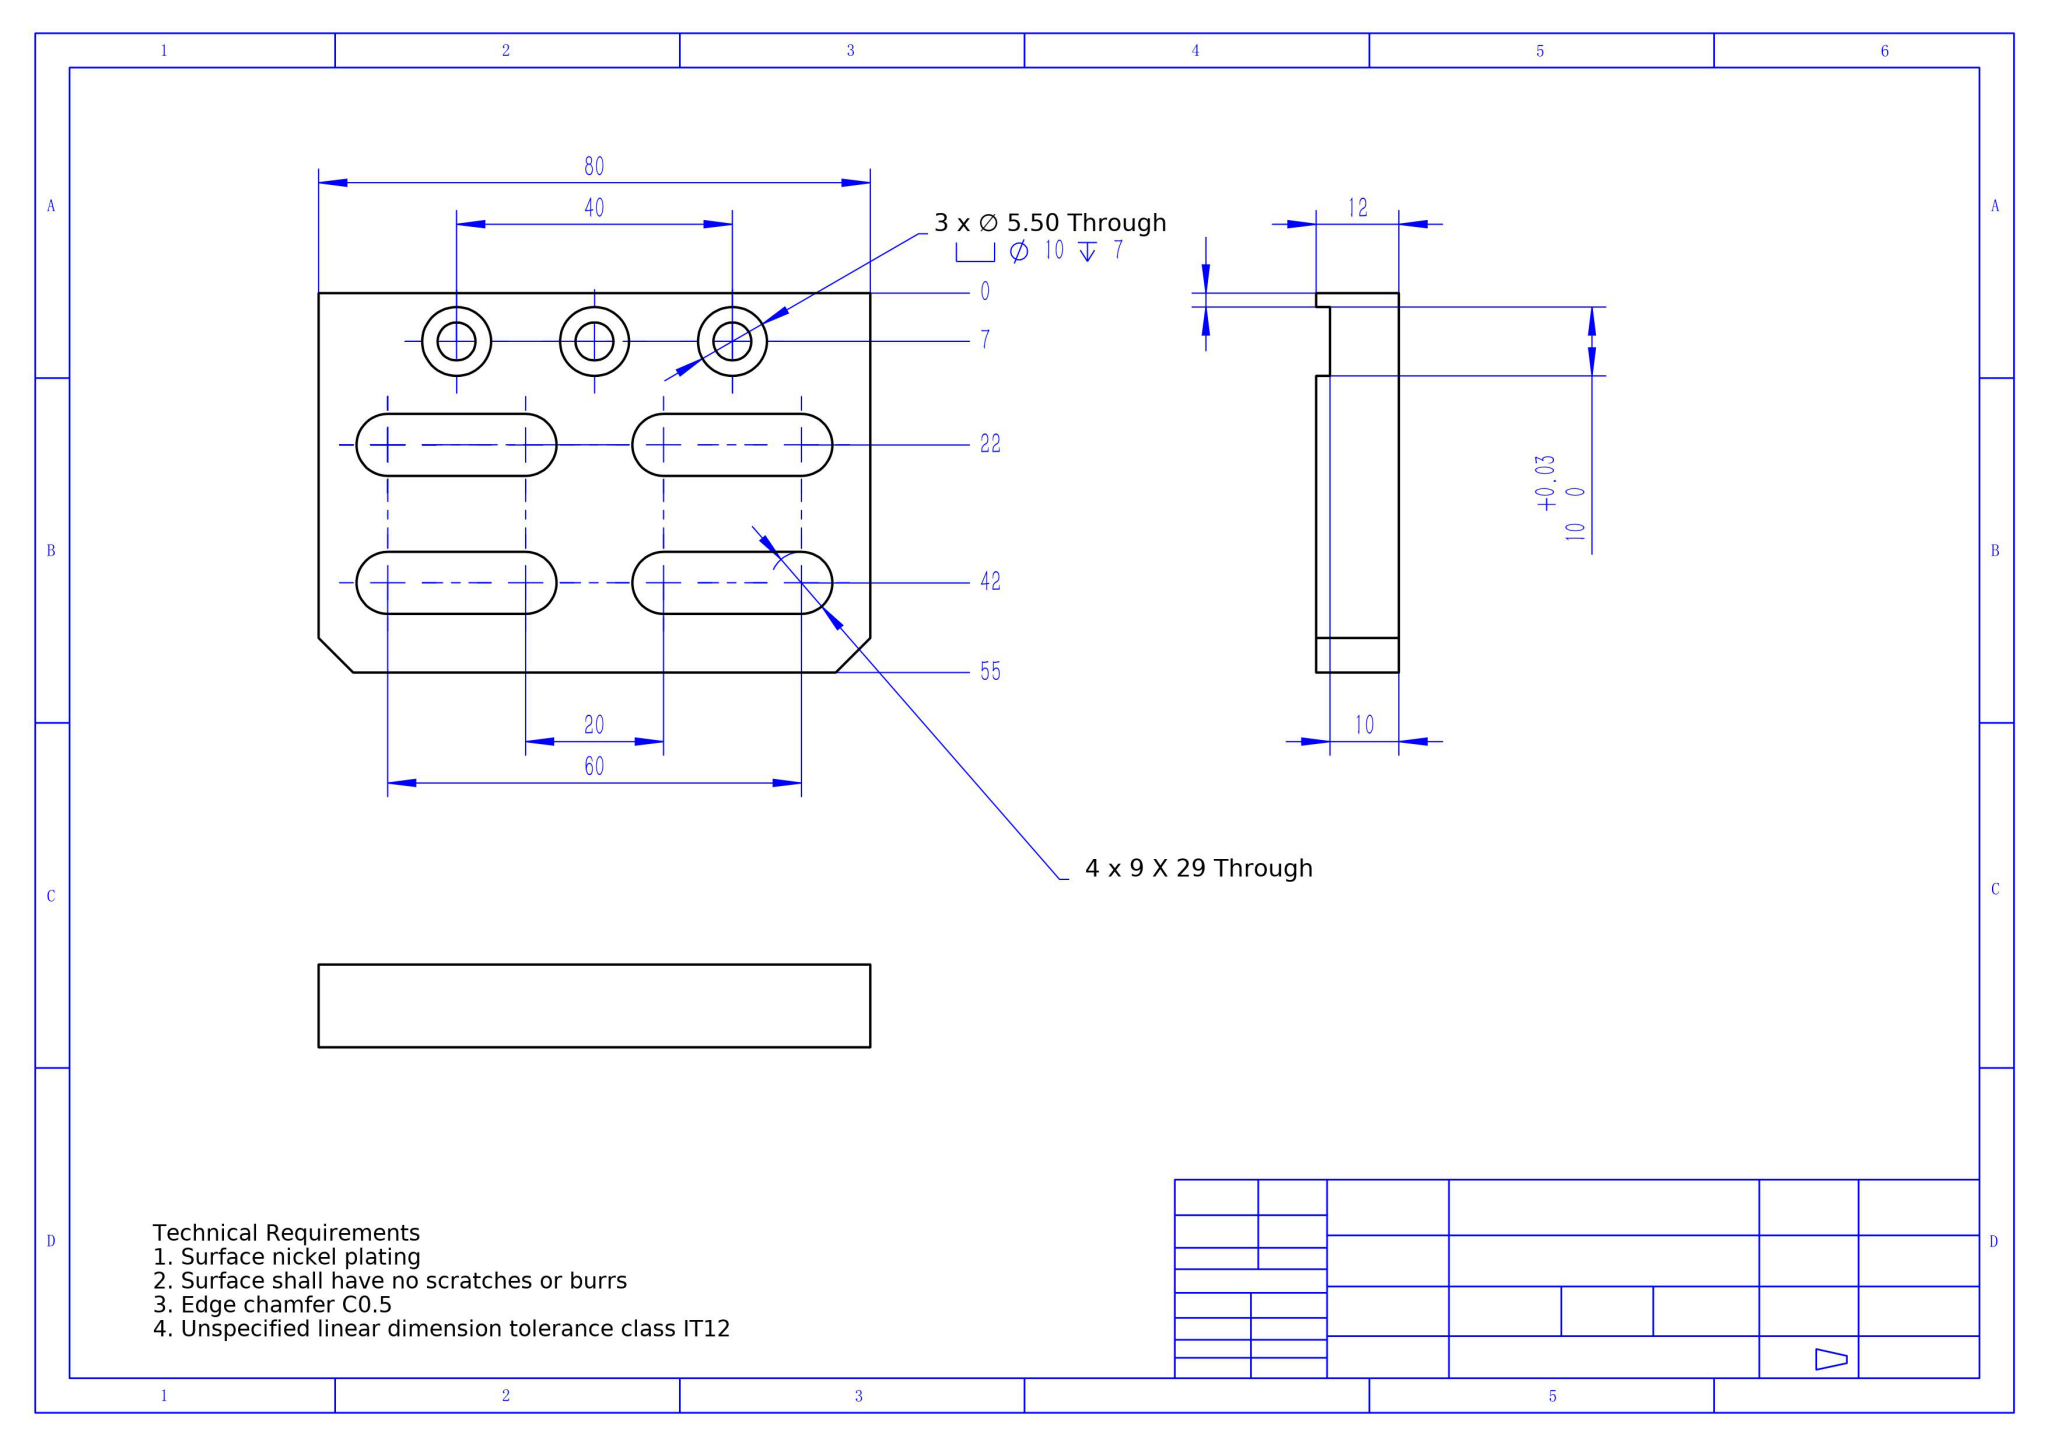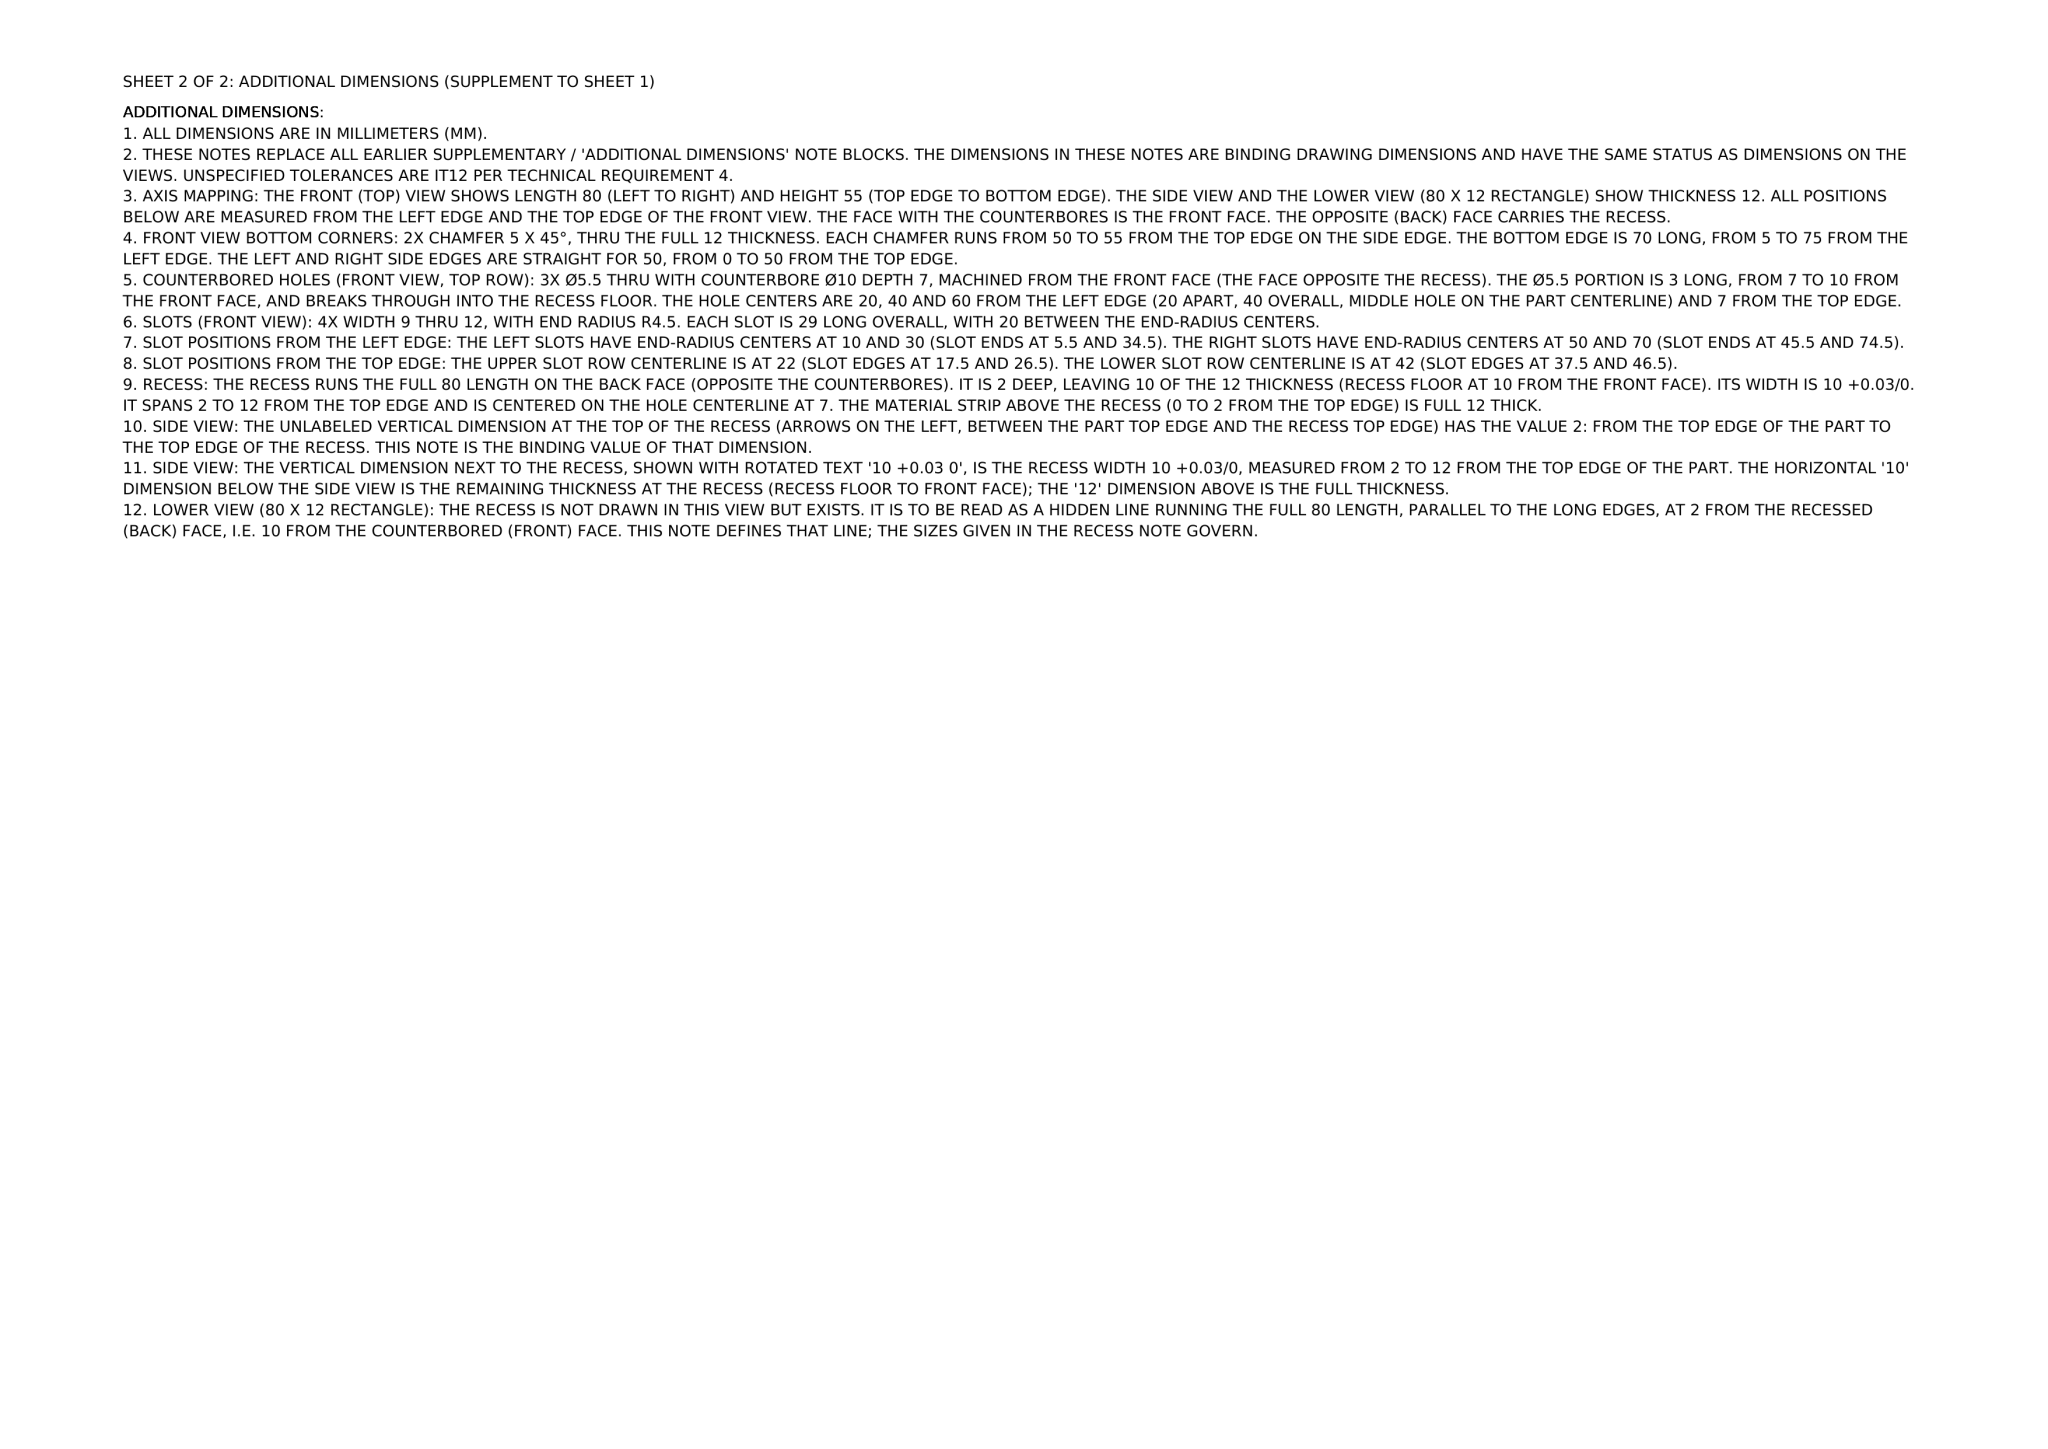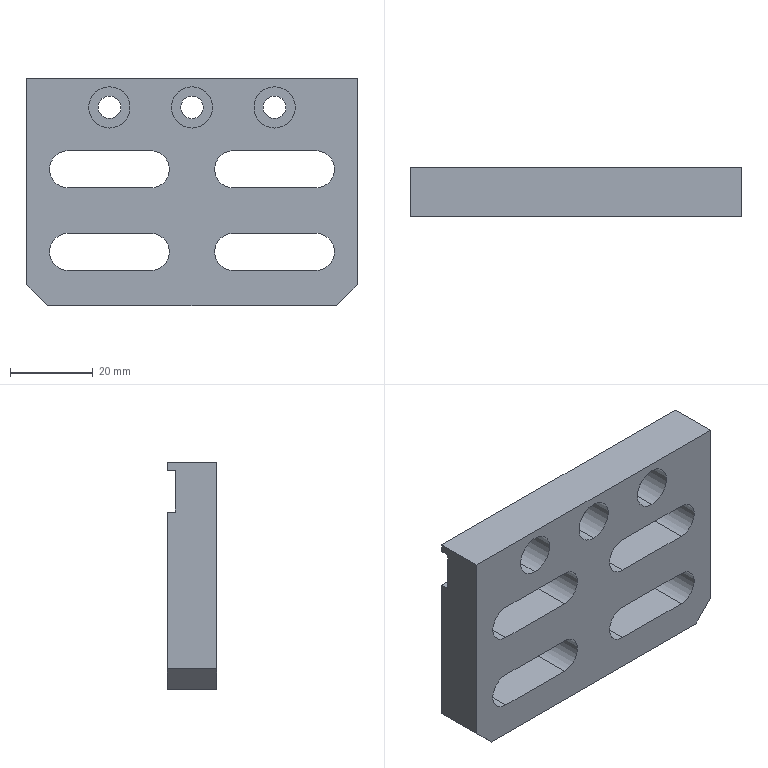Part | NX | mm | 1 solid | 43 faces | box 80 x 12 x 55 mm | volume 37343 mm3 | plane 23 | cylinder 20 | commonest cylinder face diameters 9 x8 10 x6 5.5 x6